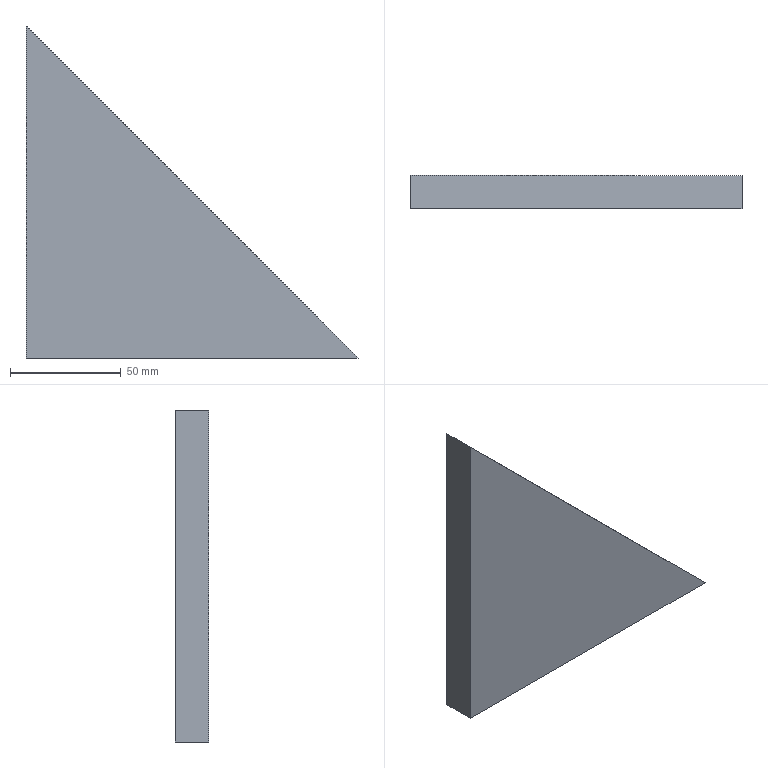Component | SolidWorks | STE21014.01-46-1 | 1 solid | 5 faces | box 150 x 15 x 150 mm | volume 168750 mm3 | plane 5 | material Q235
build123d program:
from build123d import *

# Parameters (mm, degrees)
BOSS_EXTRUDE1_DEPTH = 15


with BuildPart() as part:
    # Sketch1 → Boss-Extrude1 (new body)
    with BuildSketch(Plane(origin=(0, 0, 0), x_dir=(1, 0, 0), z_dir=(0, 1, 0))):
        Polygon((0, 0), (150, 0), (0, 150), align=None)
    extrude(amount=BOSS_EXTRUDE1_DEPTH)


solid = part.part

# Placed as in the assembly
solid = solid.moved(Location((445, 492.5, -550), (0, -90, 0)))
STEP:
#1=COLOUR_RGB('',0.7922,0.8196,0.9333);
#2=FILL_AREA_STYLE_COLOUR('',#1);
#3=FILL_AREA_STYLE('',(#2));
#4=SURFACE_STYLE_FILL_AREA(#3);
#5=SURFACE_SIDE_STYLE('',(#4));
#6=SURFACE_STYLE_USAGE(.BOTH.,#5);
#7=PRESENTATION_STYLE_ASSIGNMENT((#6));
#8=CARTESIAN_POINT('',(23.425,19.39,-21.654));
#9=VERTEX_POINT('',#8);
#10=CARTESIAN_POINT('',(17.52,19.39,-21.654));
#11=VERTEX_POINT('',#10);
#12=CARTESIAN_POINT('',(17.52,19.39,-21.654));
#13=DIRECTION('',(-1.,-0.,-0.));
#14=VECTOR('',#13,39.37);
#15=LINE('',#12,#14);
#16=EDGE_CURVE('',#9,#11,#15,.T.);
#17=ORIENTED_EDGE('',*,*,#16,.T.);
#18=CARTESIAN_POINT('',(17.52,19.98,-21.654));
#19=VERTEX_POINT('',#18);
#20=CARTESIAN_POINT('',(17.52,19.98,-21.654));
#21=DIRECTION('',(0.,-1.,0.));
#22=VECTOR('',#21,39.37);
#23=LINE('',#20,#22);
#24=EDGE_CURVE('',#19,#11,#23,.T.);
#25=ORIENTED_EDGE('',*,*,#24,.F.);
#26=CARTESIAN_POINT('',(23.425,19.98,-21.654));
#27=VERTEX_POINT('',#26);
#28=CARTESIAN_POINT('',(17.52,19.98,-21.654));
#29=DIRECTION('',(-1.,-0.,-0.));
#30=VECTOR('',#29,39.37);
#31=LINE('',#28,#30);
#32=EDGE_CURVE('',#27,#19,#31,.T.);
#33=ORIENTED_EDGE('',*,*,#32,.F.);
#34=CARTESIAN_POINT('',(23.425,19.98,-21.654));
#35=DIRECTION('',(0.,-1.,0.));
#36=VECTOR('',#35,39.37);
#37=LINE('',#34,#36);
#38=EDGE_CURVE('',#27,#9,#37,.T.);
#39=ORIENTED_EDGE('',*,*,#38,.T.);
#40=EDGE_LOOP('',(#17,#25,#33,#39));
#41=FACE_OUTER_BOUND('',#40,.T.);
#42=CARTESIAN_POINT('',(17.52,19.98,-21.654));
#43=DIRECTION('',(-0.,0.,1.));
#44=DIRECTION('',(1.,0.,0.));
#45=AXIS2_PLACEMENT_3D('',#42,#43,#44);
#46=PLANE('',#45);
#47=ADVANCED_FACE('',(#41),#46,.F.);
#48=CARTESIAN_POINT('',(17.52,19.39,-15.748));
#49=VERTEX_POINT('',#48);
#50=CARTESIAN_POINT('',(17.52,19.39,-21.654));
#51=DIRECTION('',(-0.,0.,1.));
#52=VECTOR('',#51,39.37);
#53=LINE('',#50,#52);
#54=EDGE_CURVE('',#11,#49,#53,.T.);
#55=ORIENTED_EDGE('',*,*,#54,.T.);
#56=CARTESIAN_POINT('',(17.52,19.98,-15.748));
#57=VERTEX_POINT('',#56);
#58=CARTESIAN_POINT('',(17.52,19.98,-15.748));
#59=DIRECTION('',(0.,-1.,0.));
#60=VECTOR('',#59,39.37);
#61=LINE('',#58,#60);
#62=EDGE_CURVE('',#57,#49,#61,.T.);
#63=ORIENTED_EDGE('',*,*,#62,.F.);
#64=CARTESIAN_POINT('',(17.52,19.98,-21.654));
#65=DIRECTION('',(-0.,0.,1.));
#66=VECTOR('',#65,39.37);
#67=LINE('',#64,#66);
#68=EDGE_CURVE('',#19,#57,#67,.T.);
#69=ORIENTED_EDGE('',*,*,#68,.F.);
#70=ORIENTED_EDGE('',*,*,#24,.T.);
#71=EDGE_LOOP('',(#55,#63,#69,#70));
#72=FACE_OUTER_BOUND('',#71,.T.);
#73=CARTESIAN_POINT('',(17.52,19.98,-21.654));
#74=DIRECTION('',(1.,0.,0.));
#75=DIRECTION('',(0.,-0.,-1.));
#76=AXIS2_PLACEMENT_3D('',#73,#74,#75);
#77=PLANE('',#76);
#78=ADVANCED_FACE('',(#72),#77,.F.);
#79=CARTESIAN_POINT('',(23.425,19.39,-21.654));
#80=DIRECTION('',(0.7071,-0.,-0.7071));
#81=VECTOR('',#80,39.37);
#82=LINE('',#79,#81);
#83=EDGE_CURVE('',#49,#9,#82,.T.);
#84=ORIENTED_EDGE('',*,*,#83,.T.);
#85=ORIENTED_EDGE('',*,*,#38,.F.);
#86=CARTESIAN_POINT('',(23.425,19.98,-21.654));
#87=DIRECTION('',(0.7071,-0.,-0.7071));
#88=VECTOR('',#87,39.37);
#89=LINE('',#86,#88);
#90=EDGE_CURVE('',#57,#27,#89,.T.);
#91=ORIENTED_EDGE('',*,*,#90,.F.);
#92=ORIENTED_EDGE('',*,*,#62,.T.);
#93=EDGE_LOOP('',(#84,#85,#91,#92));
#94=FACE_OUTER_BOUND('',#93,.T.);
#95=CARTESIAN_POINT('',(23.425,19.98,-21.654));
#96=DIRECTION('',(-0.7071,-0.,-0.7071));
#97=DIRECTION('',(-0.7071,0.,0.7071));
#98=AXIS2_PLACEMENT_3D('',#95,#96,#97);
#99=PLANE('',#98);
#100=ADVANCED_FACE('',(#94),#99,.F.);
#101=ORIENTED_EDGE('',*,*,#32,.T.);
#102=ORIENTED_EDGE('',*,*,#68,.T.);
#103=ORIENTED_EDGE('',*,*,#90,.T.);
#104=EDGE_LOOP('',(#101,#102,#103));
#105=FACE_OUTER_BOUND('',#104,.T.);
#106=CARTESIAN_POINT('',(17.52,19.98,-21.654));
#107=DIRECTION('',(0.,-1.,0.));
#108=DIRECTION('',(1.,0.,0.));
#109=AXIS2_PLACEMENT_3D('',#106,#107,#108);
#110=PLANE('',#109);
#111=ADVANCED_FACE('',(#105),#110,.F.);
#112=ORIENTED_EDGE('',*,*,#16,.F.);
#113=ORIENTED_EDGE('',*,*,#83,.F.);
#114=ORIENTED_EDGE('',*,*,#54,.F.);
#115=EDGE_LOOP('',(#112,#113,#114));
#116=FACE_OUTER_BOUND('',#115,.T.);
#117=CARTESIAN_POINT('',(17.52,19.39,-21.654));
#118=DIRECTION('',(0.,-1.,0.));
#119=DIRECTION('',(1.,0.,0.));
#120=AXIS2_PLACEMENT_3D('',#117,#118,#119);
#121=PLANE('',#120);
#122=ADVANCED_FACE('',(#116),#121,.T.);
#123=CLOSED_SHELL('',(#47,#78,#100,#111,#122));
#124=MANIFOLD_SOLID_BREP('',#123);
#125=STYLED_ITEM('',(#7),#124);
#126=PRESENTATION_LAYER_ASSIGNMENT('','',(#125));
#127=CARTESIAN_POINT('',(0.,0.,0.));
#128=DIRECTION('',(0.,0.,1.));
#129=DIRECTION('',(1.,0.,0.));
#130=AXIS2_PLACEMENT_3D('',#127,#128,#129);
#131=(LENGTH_UNIT()NAMED_UNIT(*)SI_UNIT($,.METRE.));
#132=LENGTH_MEASURE_WITH_UNIT(LENGTH_MEASURE(0.0254),#131);
#133=DIMENSIONAL_EXPONENTS(1.,0.,0.,0.,0.,0.,0.);
#134=(CONVERSION_BASED_UNIT('',#132)LENGTH_UNIT()NAMED_UNIT(#133));
#135=UNCERTAINTY_MEASURE_WITH_UNIT(LENGTH_MEASURE(0.00001),#134,'','');
#136=(NAMED_UNIT(*)PLANE_ANGLE_UNIT()SI_UNIT($,.RADIAN.));
#137=(NAMED_UNIT(*)SI_UNIT($,.STERADIAN.)SOLID_ANGLE_UNIT());
#138=(GEOMETRIC_REPRESENTATION_CONTEXT(3)GLOBAL_UNCERTAINTY_ASSIGNED_CONTEXT((#135))GLOBAL_UNIT_ASSIGNED_CONTEXT((#134,#136,#137))REPRESENTATION_CONTEXT('',''));
#139=ADVANCED_BREP_SHAPE_REPRESENTATION('',(#124,#130),#138);
#140=(LENGTH_UNIT()NAMED_UNIT(*)SI_UNIT($,.METRE.));
#141=LENGTH_MEASURE_WITH_UNIT(LENGTH_MEASURE(0.0254),#140);
#142=DIMENSIONAL_EXPONENTS(1.,0.,0.,0.,0.,0.,0.);
#143=(CONVERSION_BASED_UNIT('',#141)LENGTH_UNIT()NAMED_UNIT(#142));
#144=UNCERTAINTY_MEASURE_WITH_UNIT(LENGTH_MEASURE(0.00001),#143,'','');
#145=(NAMED_UNIT(*)PLANE_ANGLE_UNIT()SI_UNIT($,.RADIAN.));
#146=(NAMED_UNIT(*)SI_UNIT($,.STERADIAN.)SOLID_ANGLE_UNIT());
#147=(GEOMETRIC_REPRESENTATION_CONTEXT(3)GLOBAL_UNCERTAINTY_ASSIGNED_CONTEXT((#144))GLOBAL_UNIT_ASSIGNED_CONTEXT((#143,#145,#146))REPRESENTATION_CONTEXT('',''));
#148=MECHANICAL_DESIGN_GEOMETRIC_PRESENTATION_REPRESENTATION('',(#125),#147);